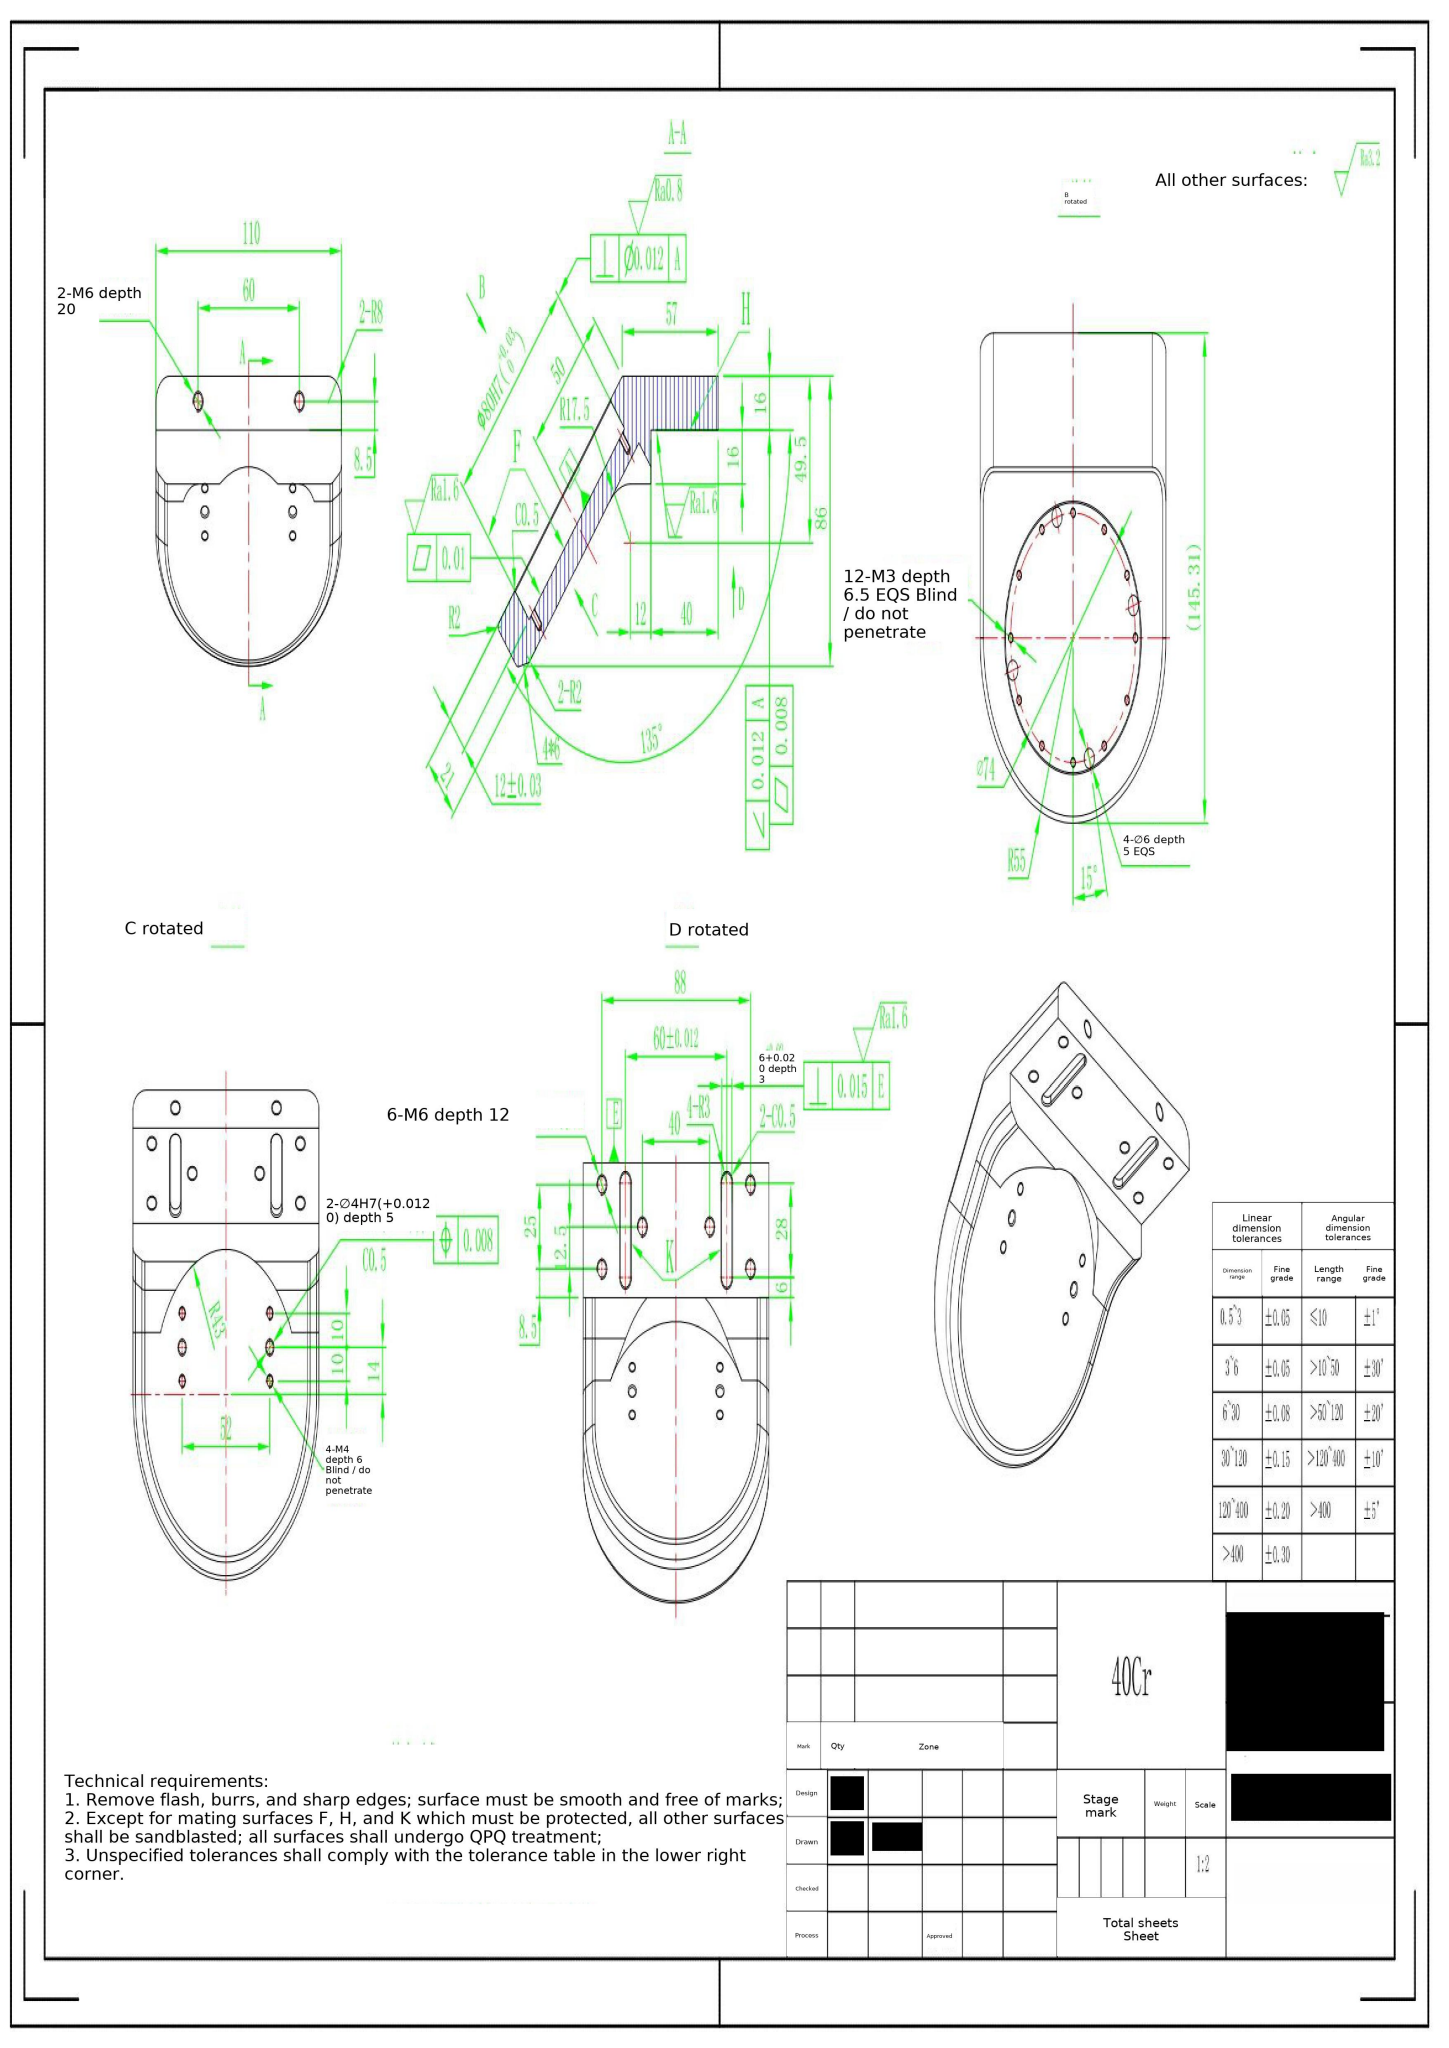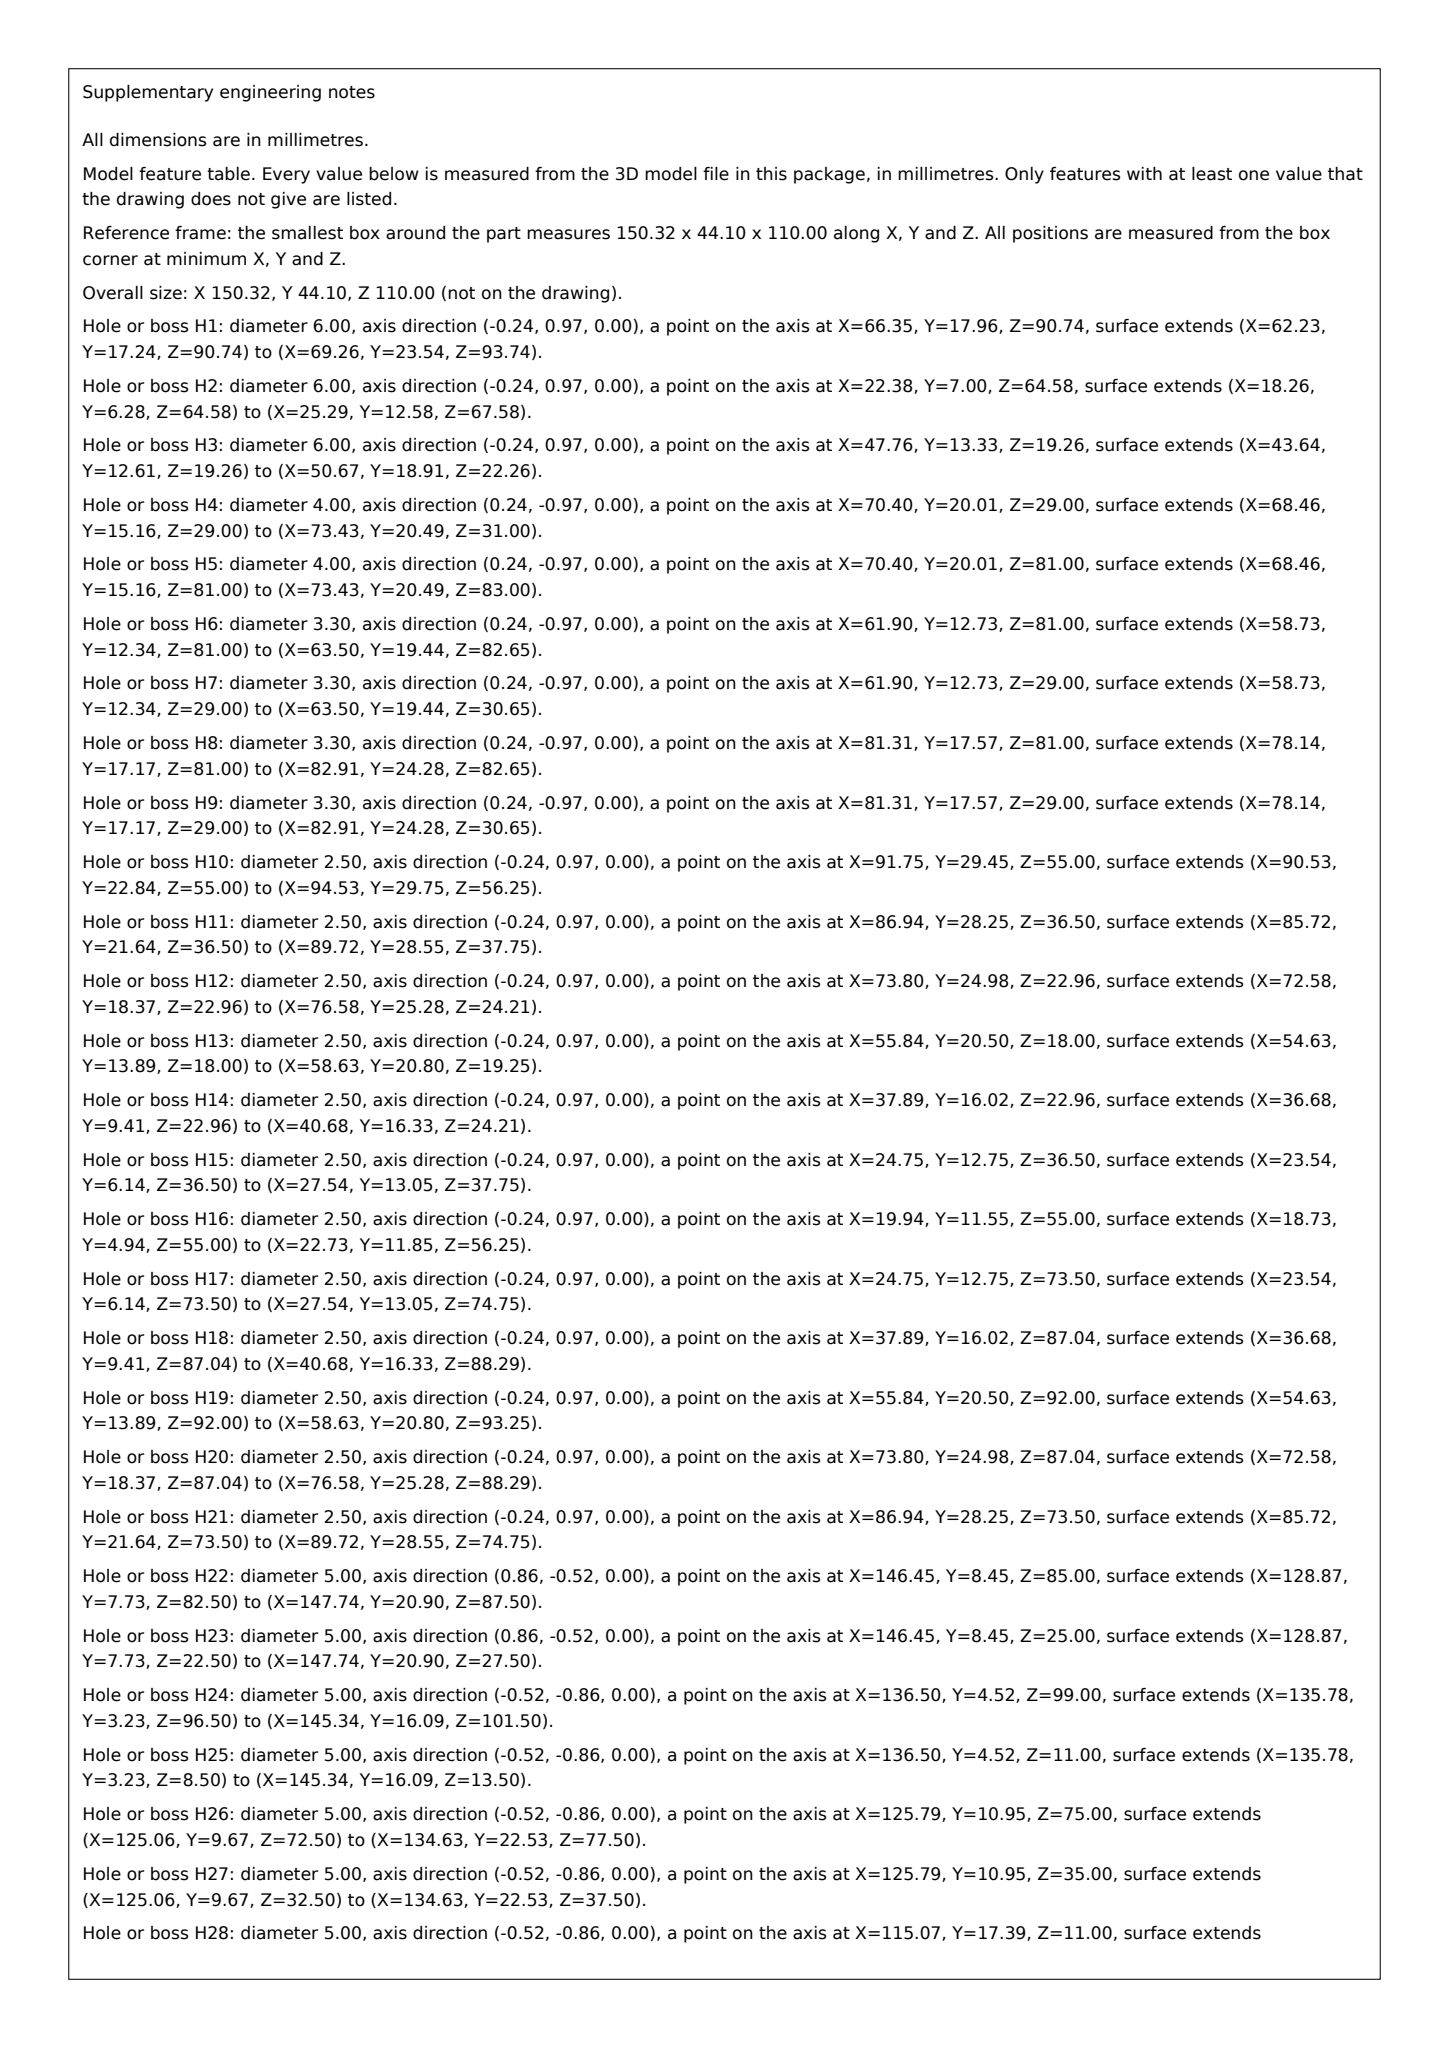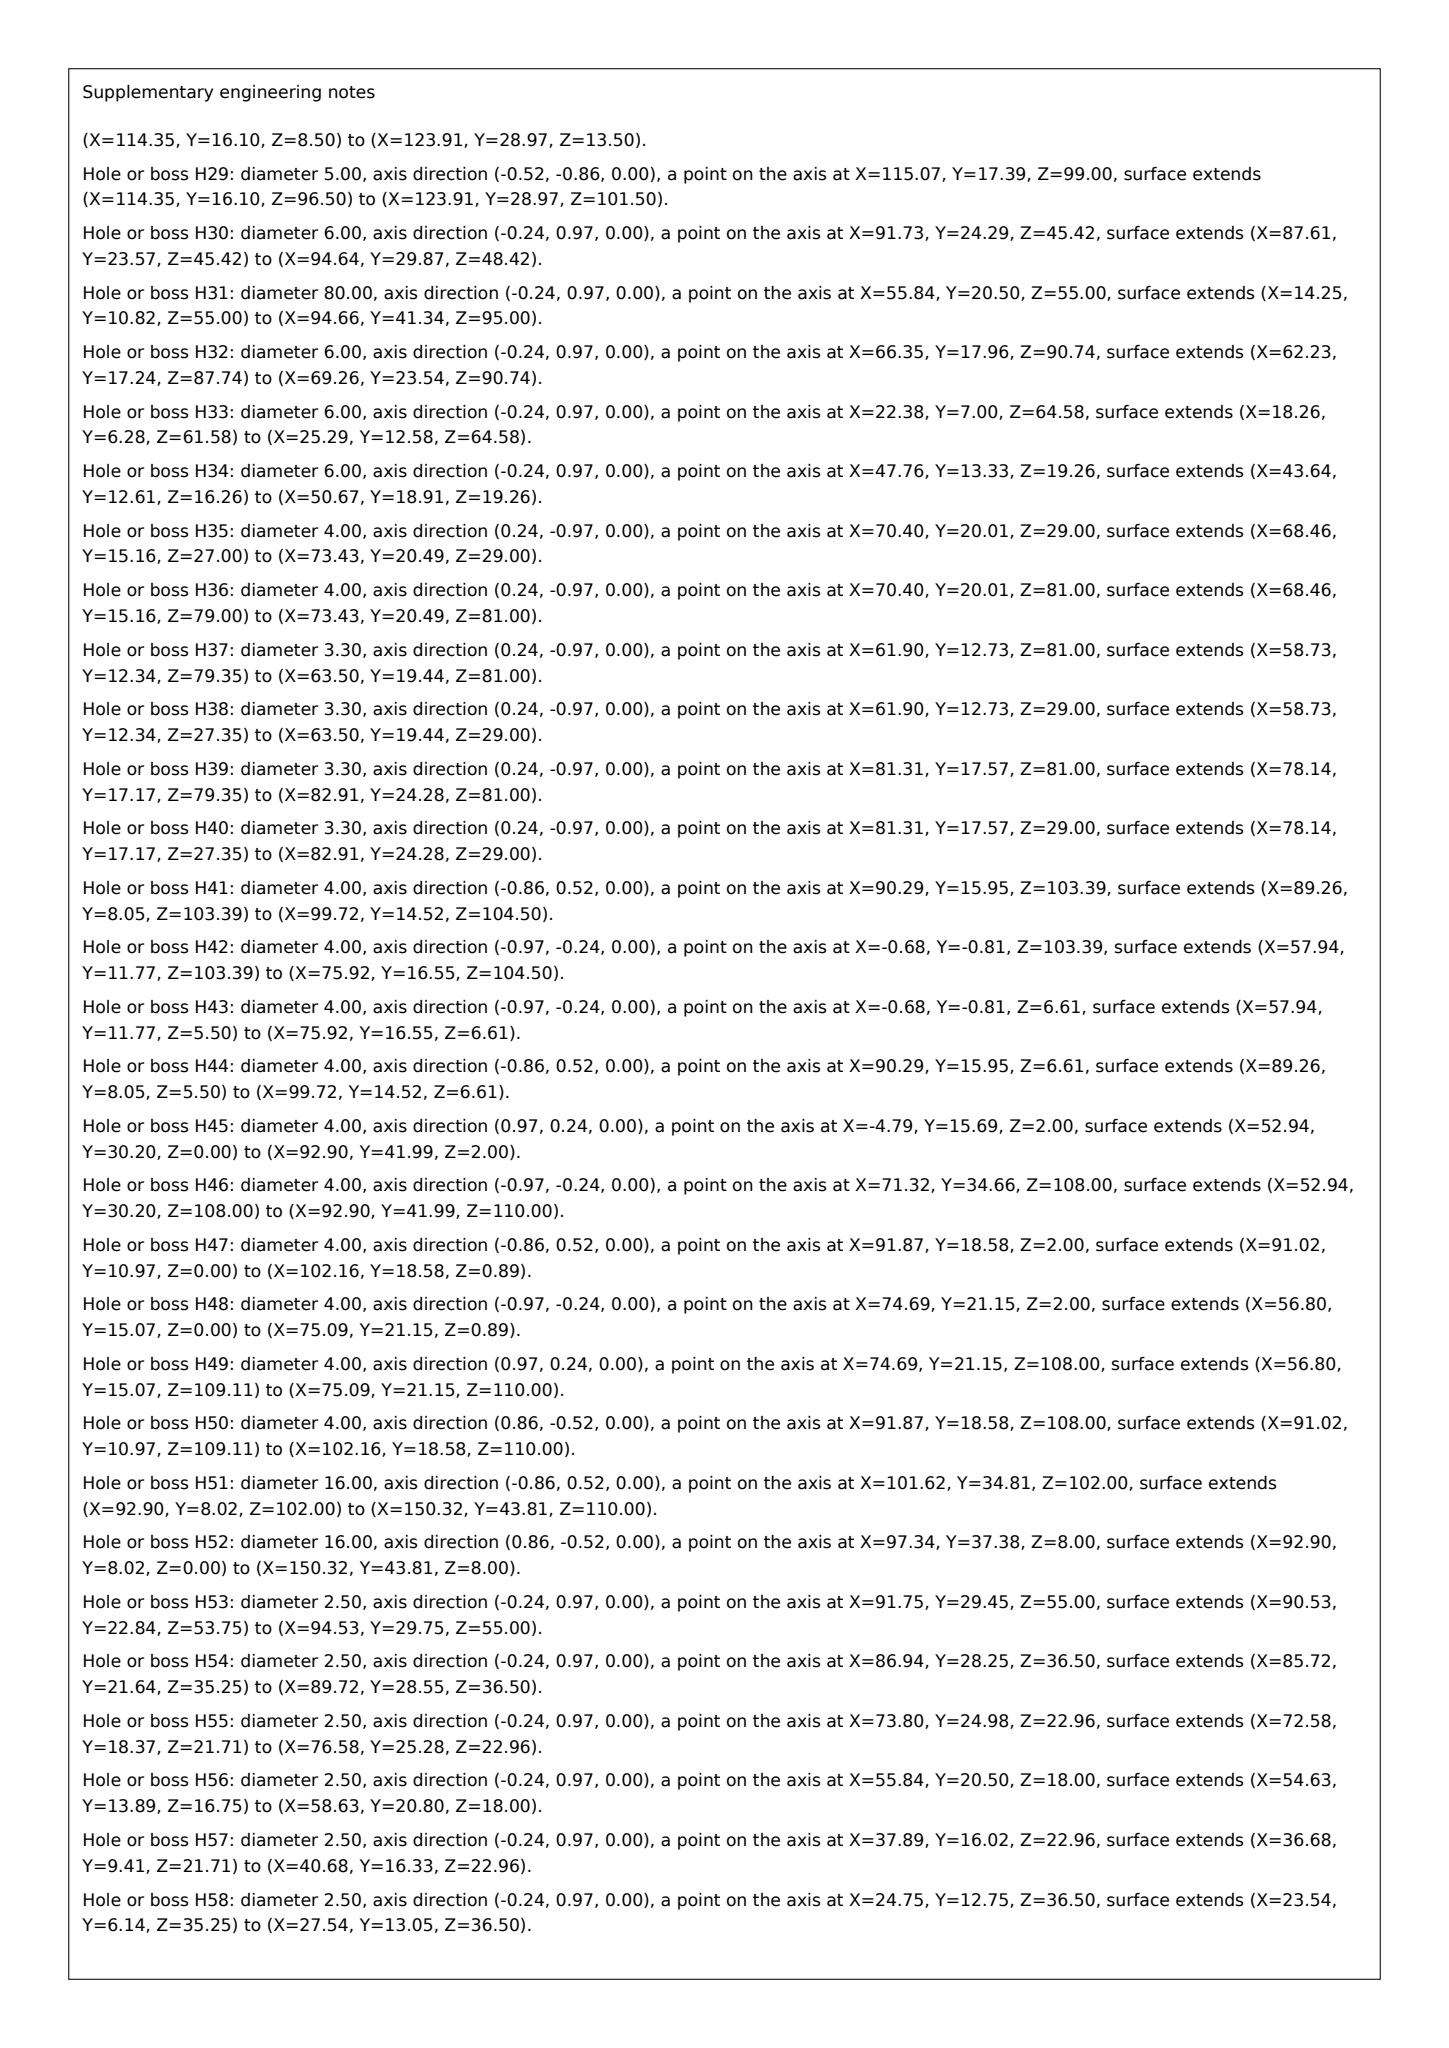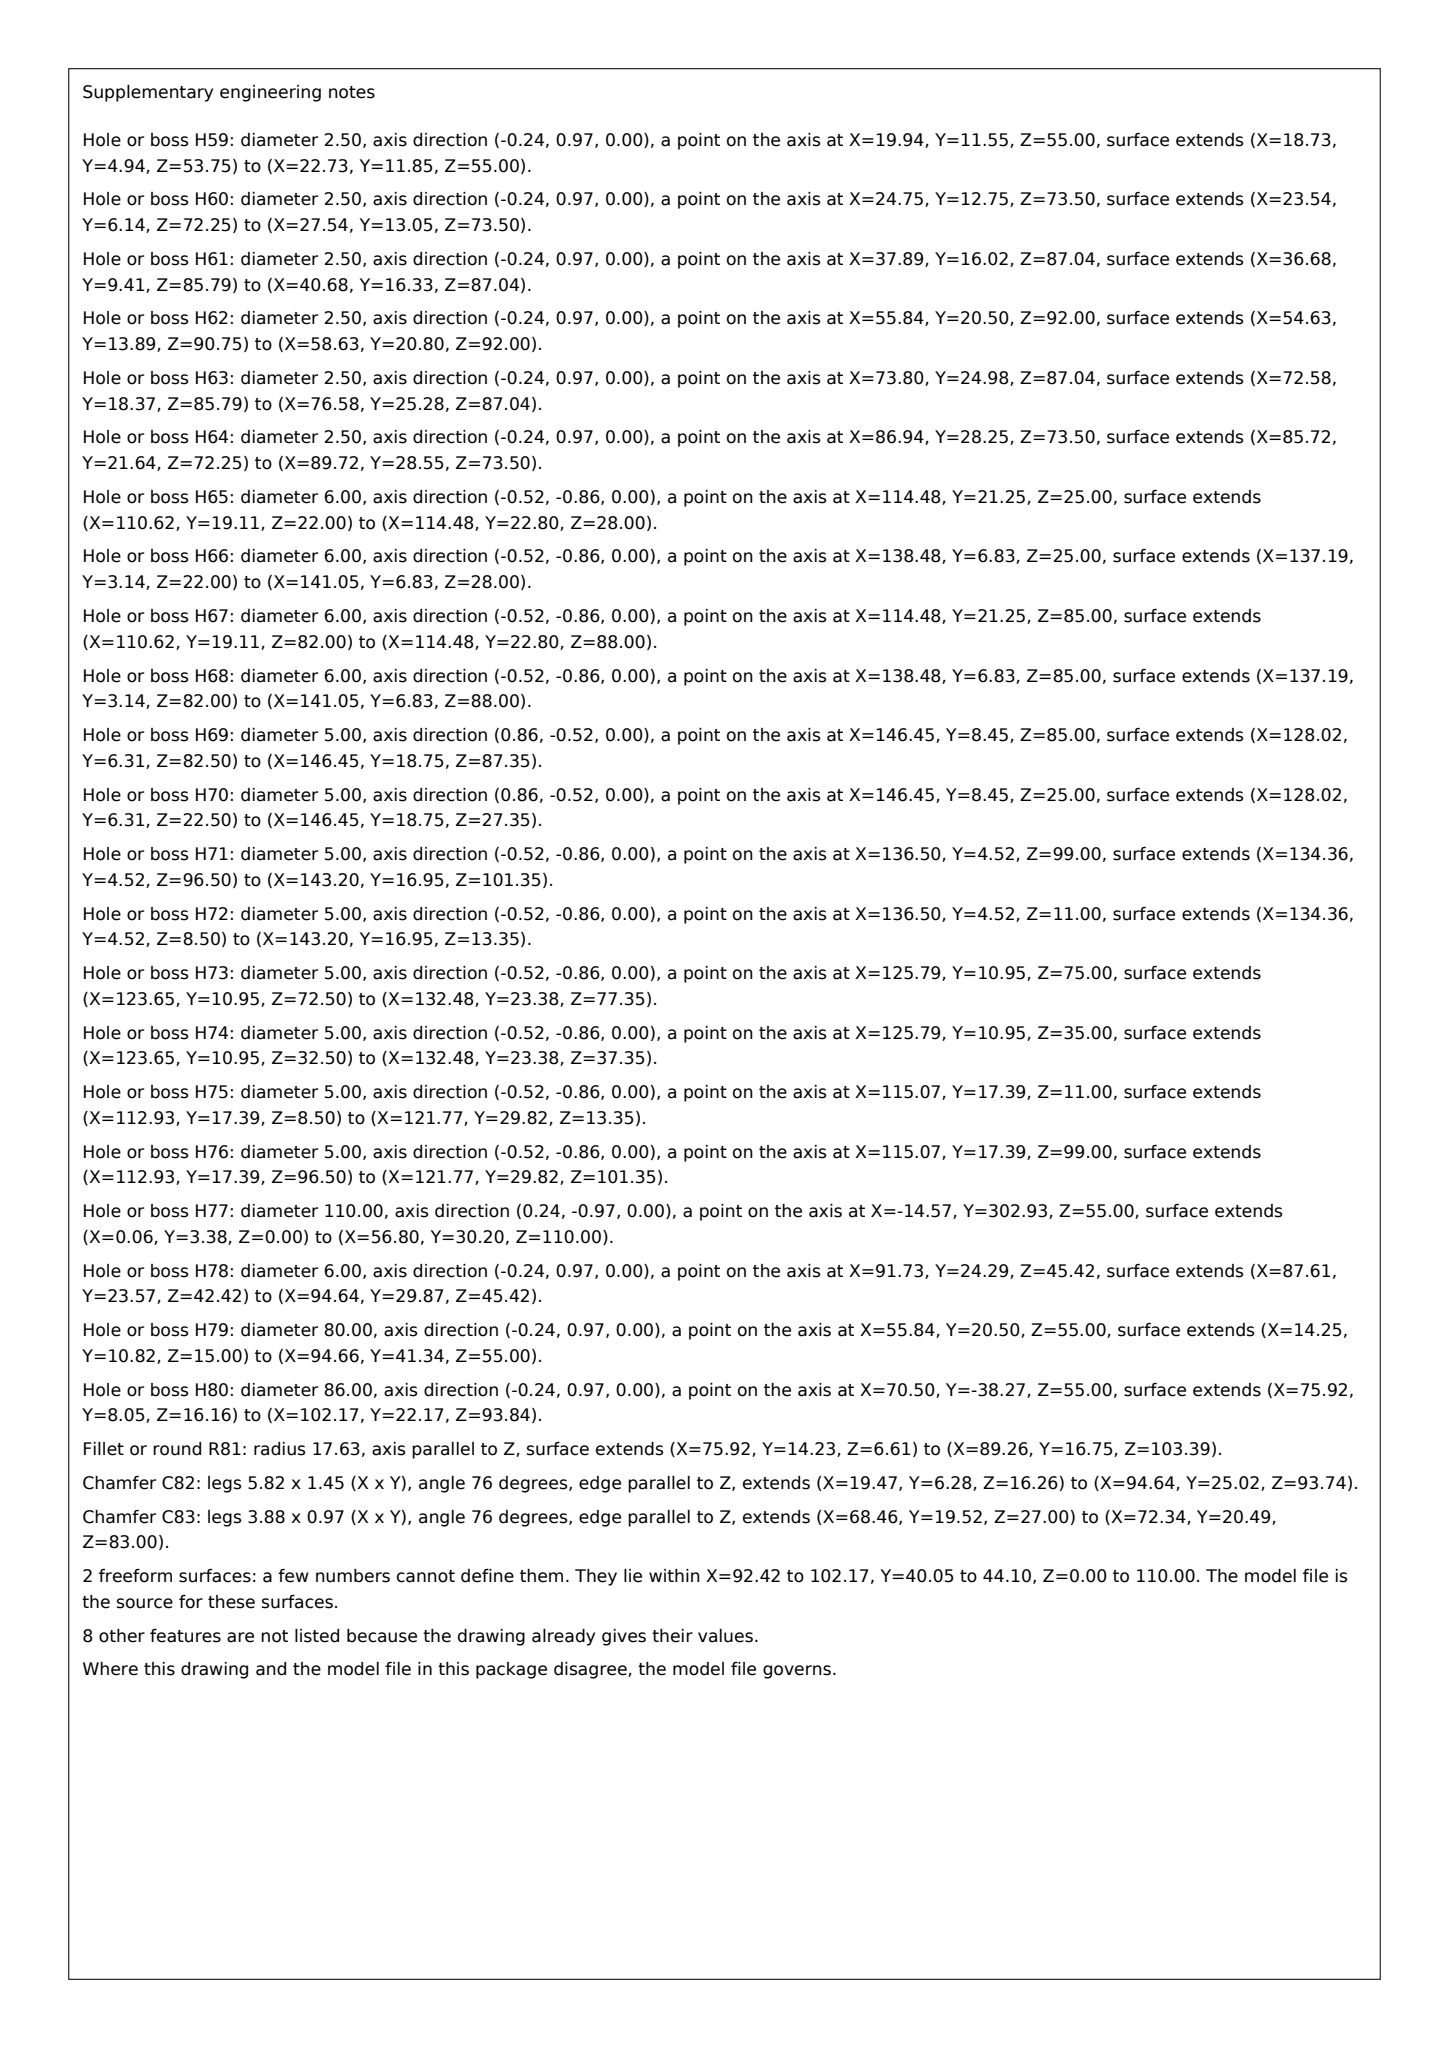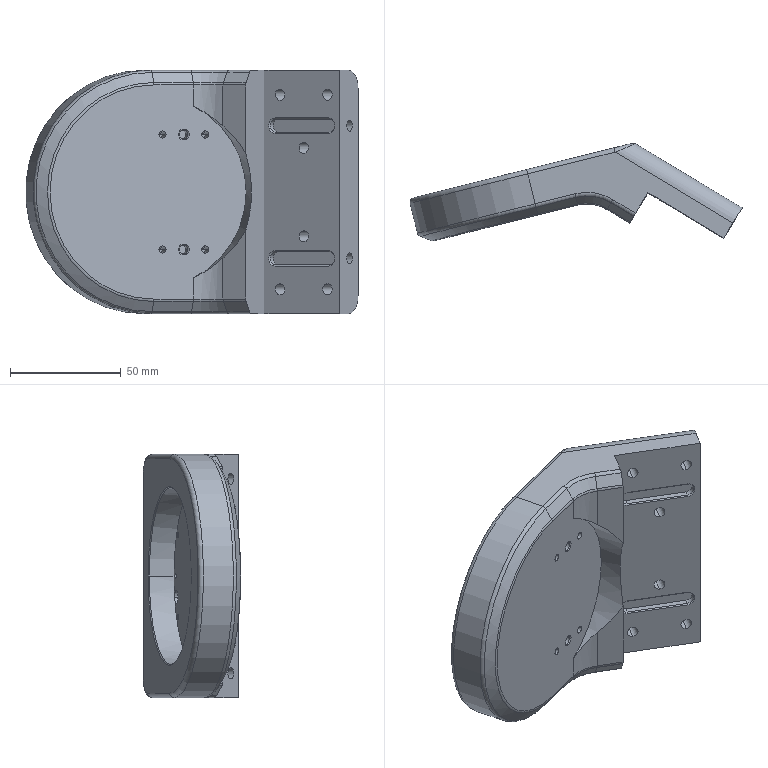Part | SolidWorks | mm | material 40Cr | 1 solid | 184 faces | box 150.32 x 44.1 x 110 mm | volume 245971 mm3 | cylinder 83 | cone 61 | plane 31 | torus 7 | spline 2 | commonest cylinder face diameters 2.5 x24 5 x16 4 x15 6 x12 3.3 x8 80 x2 16 x2 35.255 x2